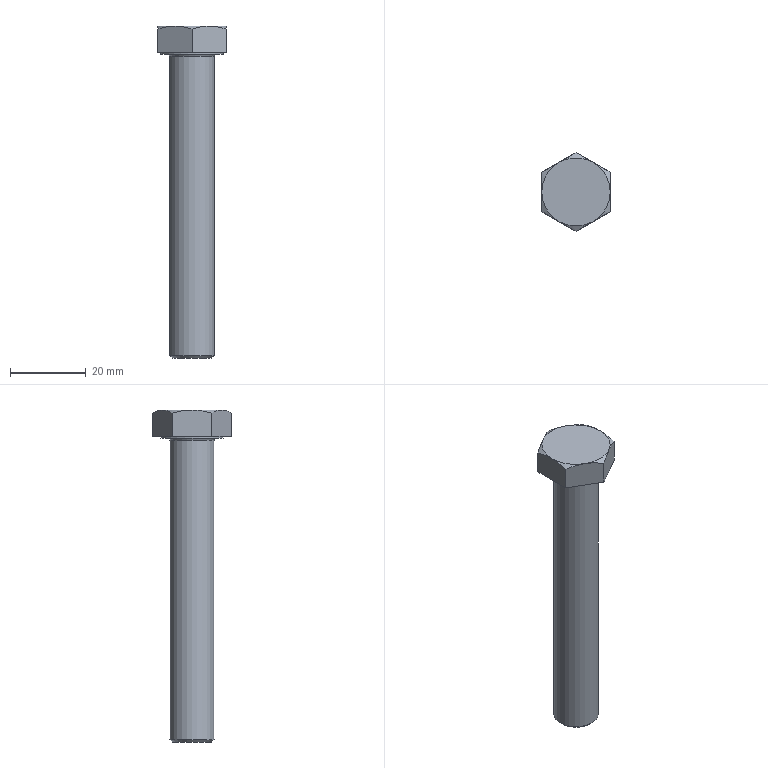Component | NX | GB-T5782-2000_M12X80_3 | 1 solid | 20 faces | volume 10657 mm3 | plane 10 | cone 7 | cylinder 2 | torus 1 | commonest cylinder face diameters 16.47 x1 11.701 x1